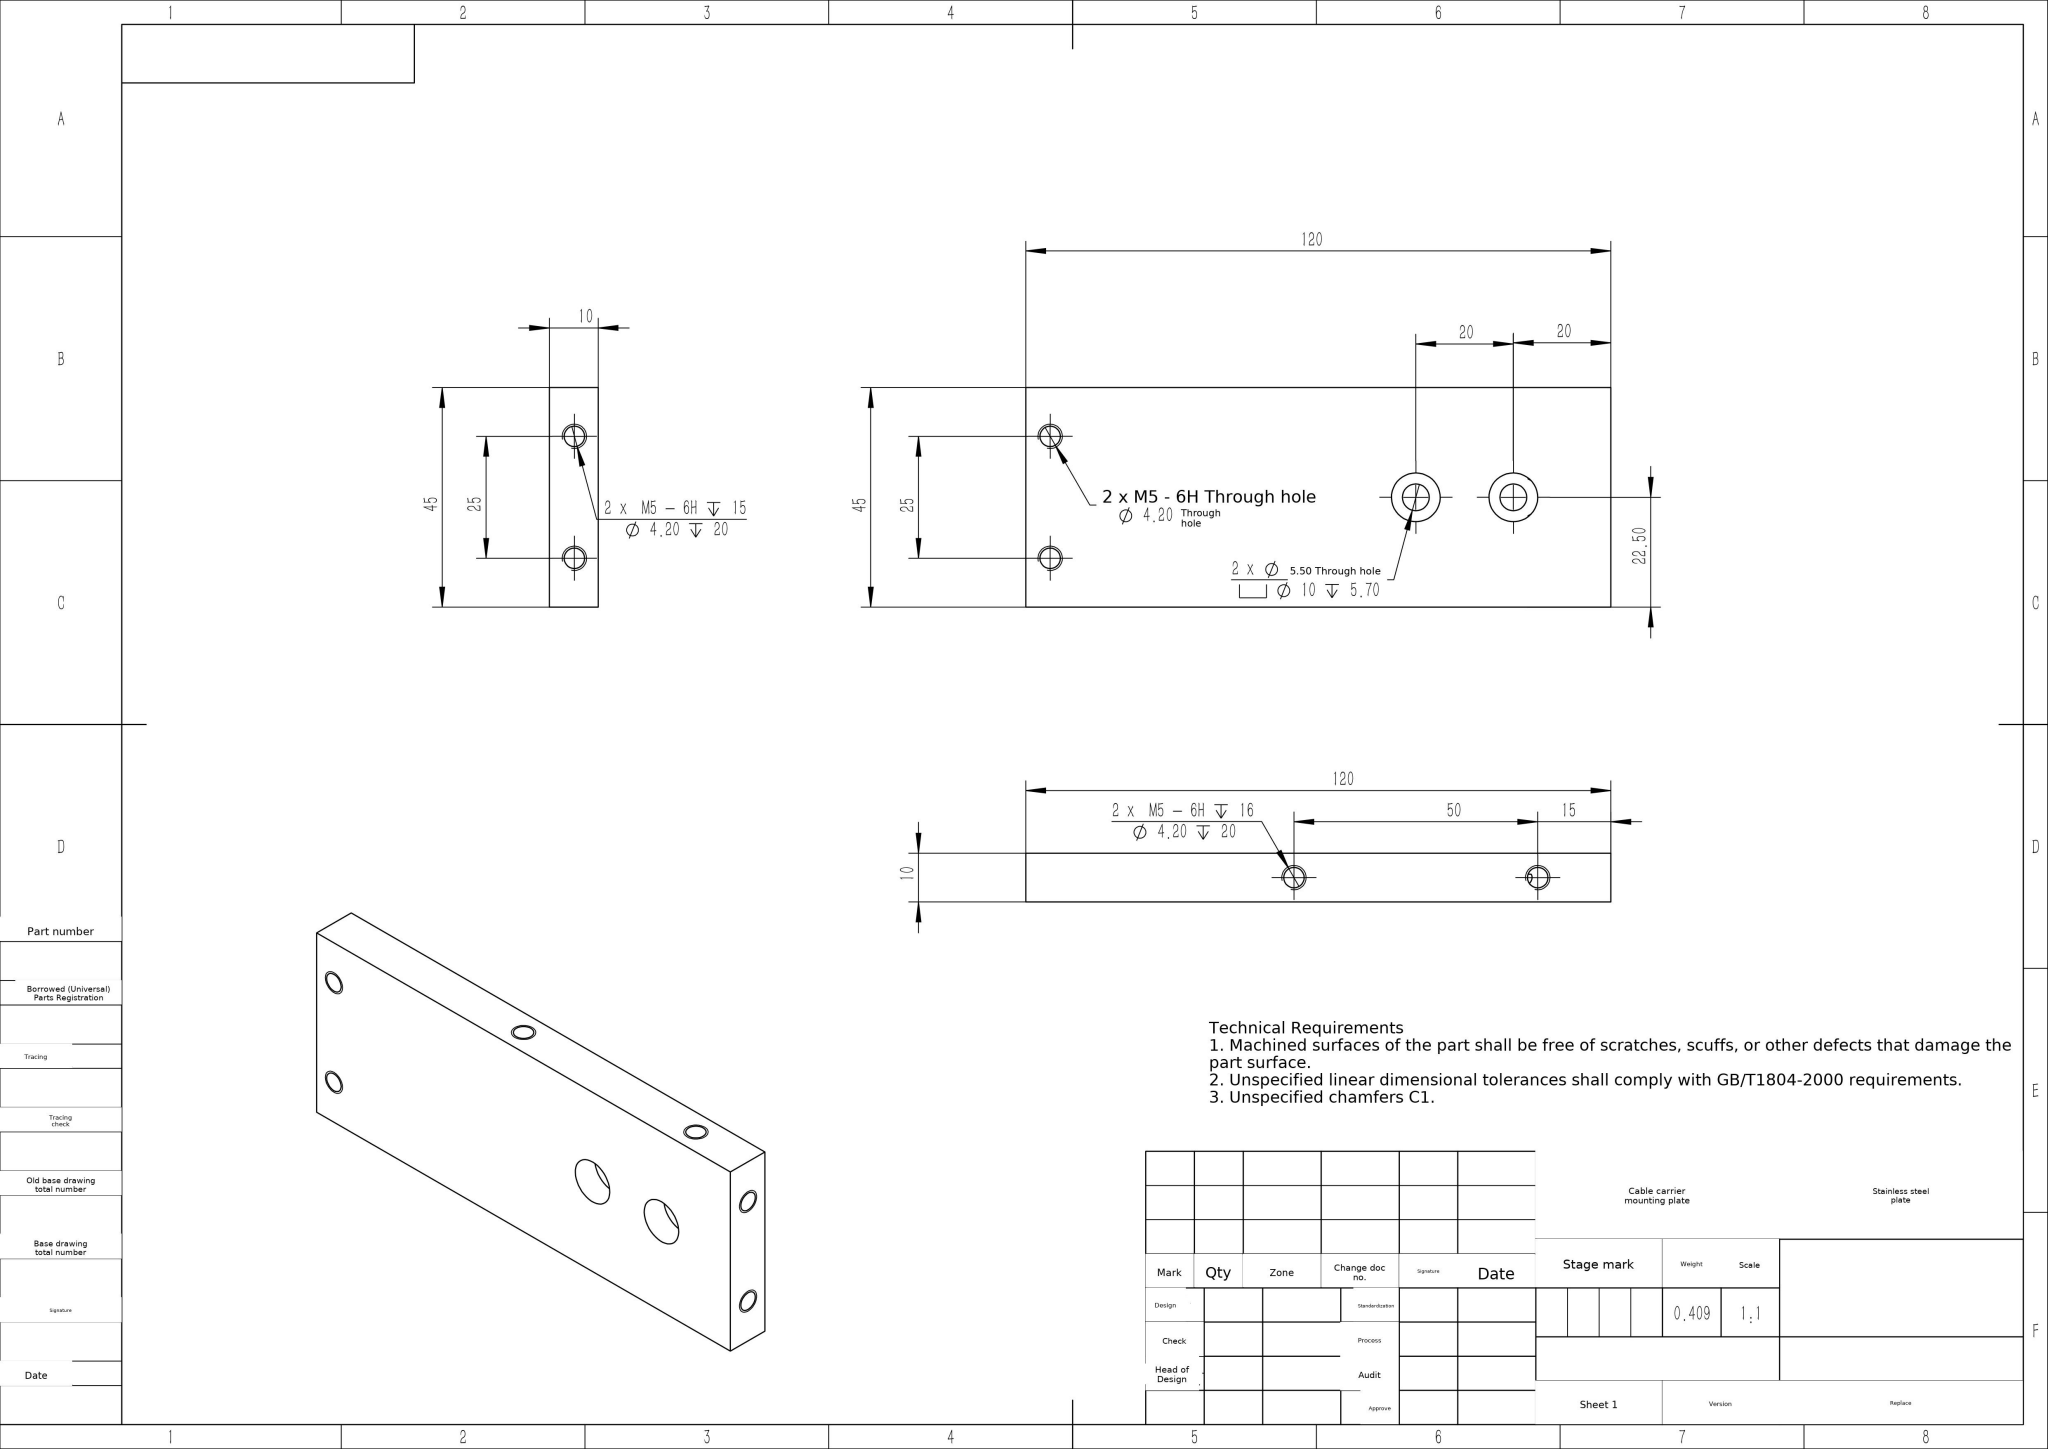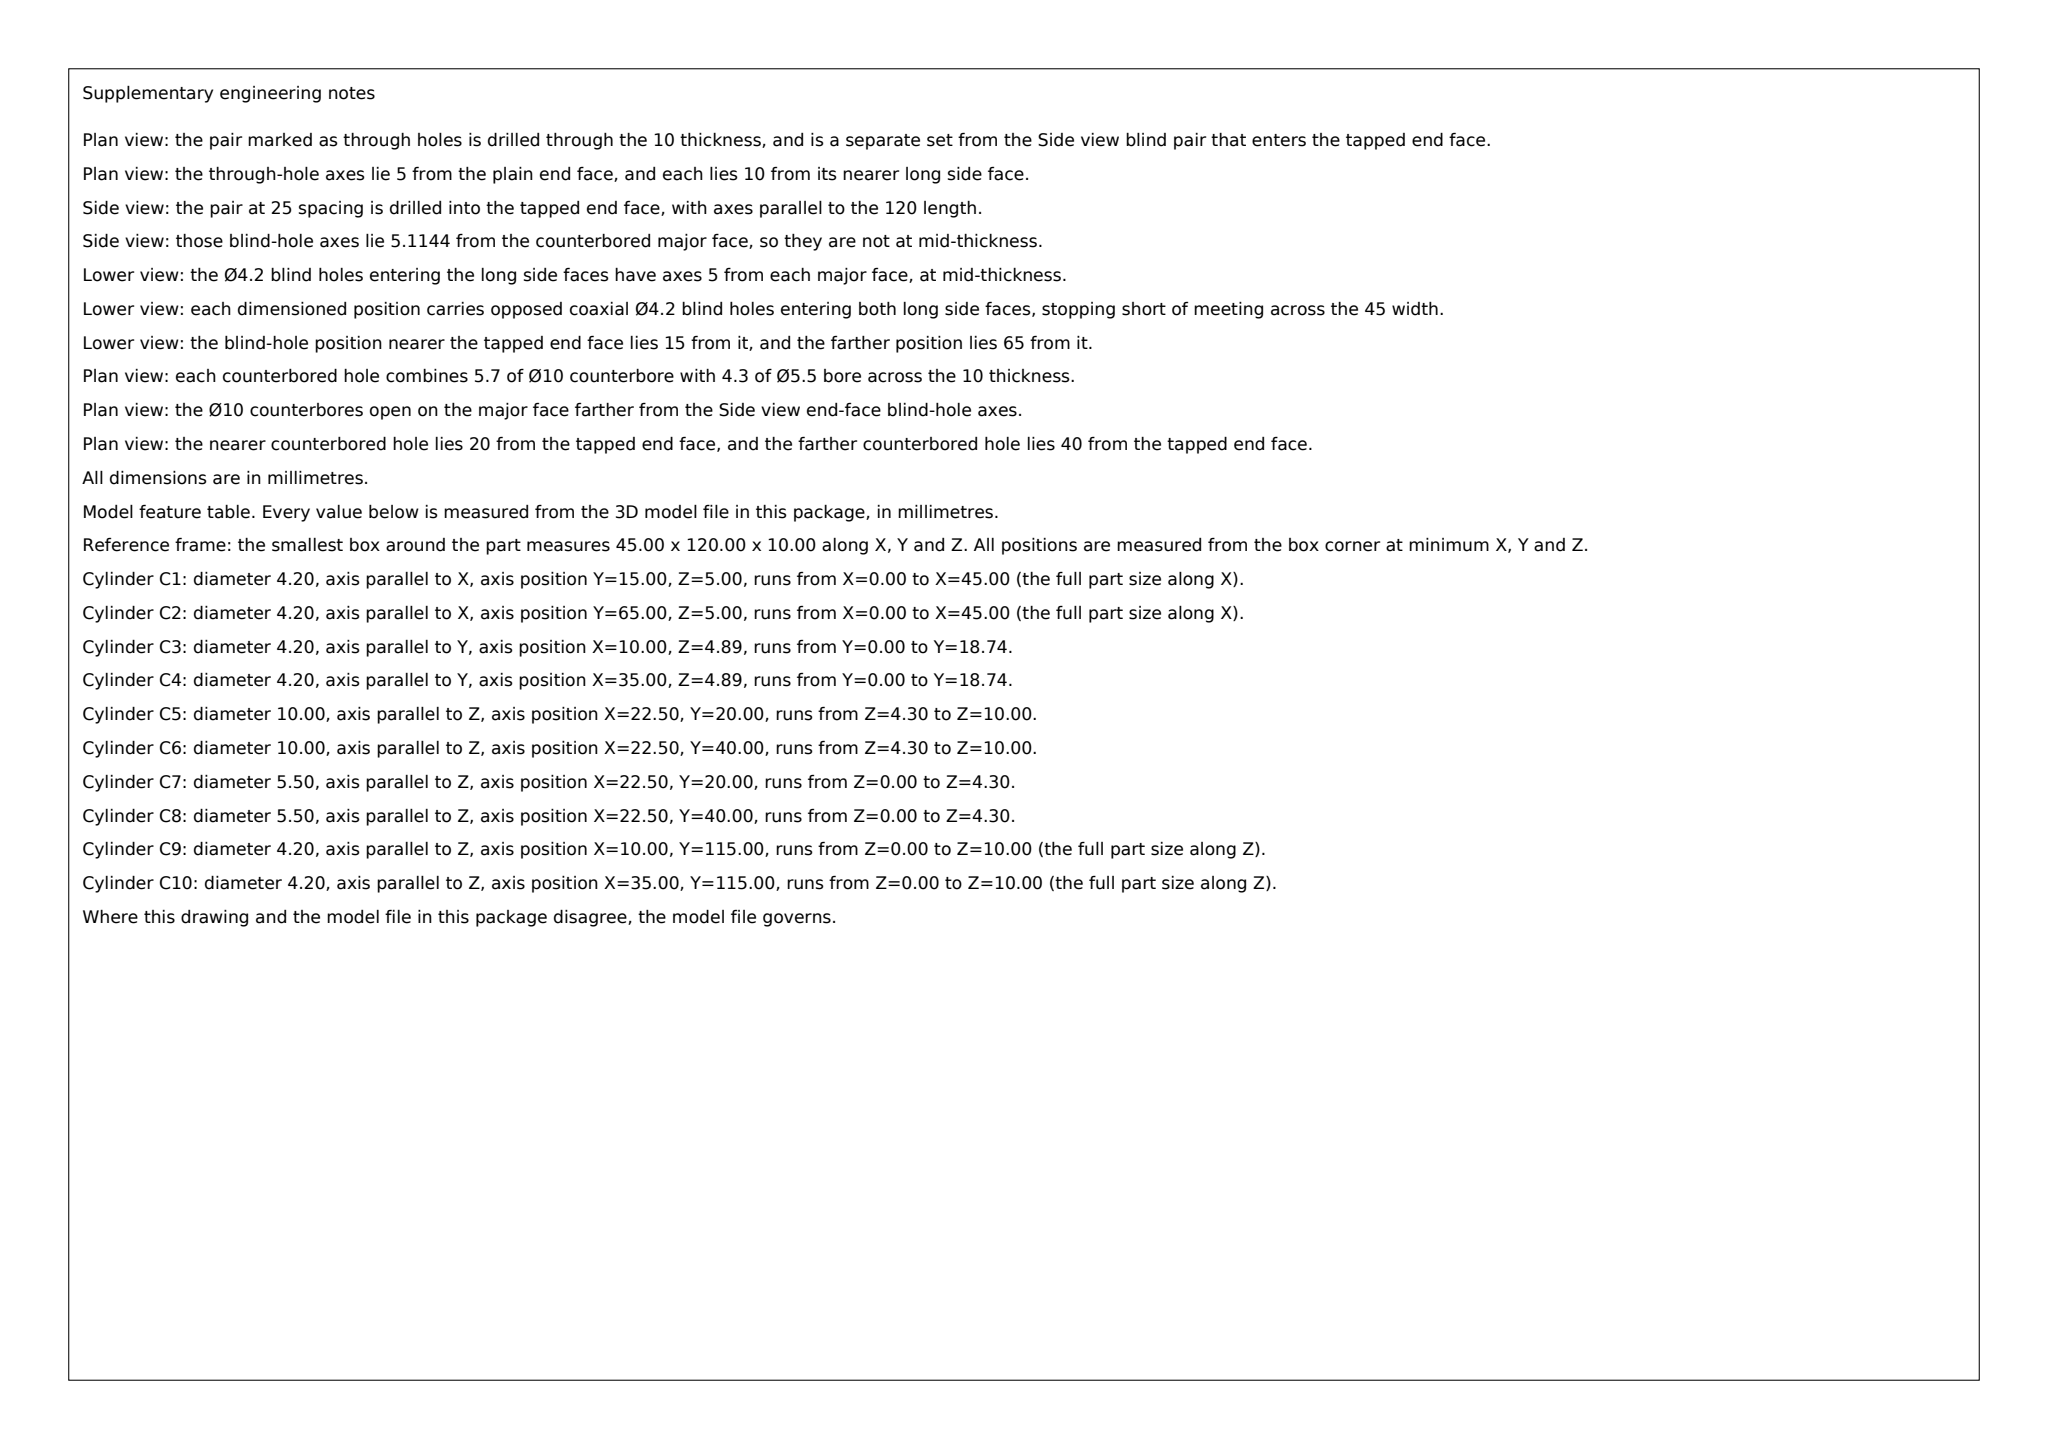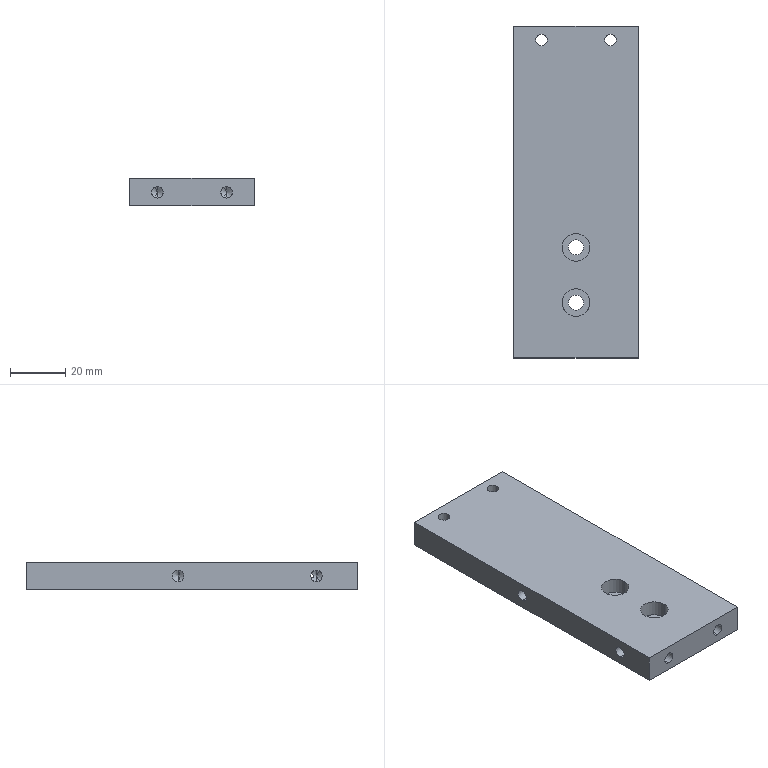Part | SolidWorks | mm | material Stainless steel plate | 1 solid | 44 faces | box 45 x 120 x 10 mm | volume 51129 mm3 | cylinder 24 | cone 12 | plane 8 | commonest cylinder face diameters 4.2 x16 5.5 x4 10 x4
Drawing notes:
OPP 120x10 FACE: 2 x M5-6H DP 16 / Ø4.20 DP 20, SAME LOCS AS SHOWN | from the solid: 4.2 dia holes, axis x, at y=15 & y=65, z=5, len 18.74 + 118 deg point; entering both x=0 and x=45 faces (4 total)
SIDE FACE TAPPED HOLES ON C/L OF 10 THK (5 FROM EA FACE) | from the solid: axis-x cylinders pos z=5.0 of 10.0 thk; y=15 & 65 (=15 & 65 from end, 50 apart)
build123d program:
from build123d import *

# Parameters (mm, degrees)
SKETCH6_W                                       = 45
SKETCH6_H                                       = 120
BOSS_EXTRUDE1_DEPTH                             = 10
M5_TAPPED_HOLE1_D                               = 4.2
M5_TAPPED_HOLE2_D                               = 4.2
M5_TAPPED_HOLE2_DEPTH                           = 18.738
M5_TAPPED_HOLE2_TIP                             = 1.262
M5_TAPPED_HOLE3_D                               = 4.2
M5_TAPPED_HOLE3_DEPTH                           = 18.738
M5_TAPPED_HOLE3_TIP                             = 1.262
M5_TAPPED_HOLE4_D                               = 4.2
M5_TAPPED_HOLE4_DEPTH                           = 18.738
M5_TAPPED_HOLE4_TIP                             = 1.262
M5_HEX_SOCKET_HEAD_CAP_SCREW_CBORE1_D           = 5.5
M5_HEX_SOCKET_HEAD_CAP_SCREW_CBORE1_CBORE_D     = 10
M5_HEX_SOCKET_HEAD_CAP_SCREW_CBORE1_CBORE_DEPTH = 5.7


with BuildPart() as part:
    # Sketch6 → Boss-Extrude1 (new body)
    with BuildSketch(Plane.XY):
        Rectangle(SKETCH6_W, SKETCH6_H)
    extrude(amount=BOSS_EXTRUDE1_DEPTH)

    # M5 Tapped Hole1 (through all)
    with Locations(Plane.XY.offset(10)):
        with Locations((12.5, 55), (-12.5, 55)):
            Hole(M5_TAPPED_HOLE1_D / 2)

    # M5 Tapped Hole2
    with Locations(Plane.ZY.offset(22.5)):
        with Locations((5, -45), (5, 5)):
            Hole(M5_TAPPED_HOLE2_D / 2, depth=M5_TAPPED_HOLE2_DEPTH)
            with Locations((0, 0, -(M5_TAPPED_HOLE2_DEPTH + M5_TAPPED_HOLE2_TIP / 2))):  # 118° drill point
                Cone(0, M5_TAPPED_HOLE2_D / 2, M5_TAPPED_HOLE2_TIP, mode=Mode.SUBTRACT)

    # M5 Tapped Hole3
    with Locations(Plane(origin=(22.5, 0, 0), x_dir=(0, 0, -1), z_dir=(1, 0, 0))):
        with Locations((-5, -45), (-5, 5)):
            Hole(M5_TAPPED_HOLE3_D / 2, depth=M5_TAPPED_HOLE3_DEPTH)
            with Locations((0, 0, -(M5_TAPPED_HOLE3_DEPTH + M5_TAPPED_HOLE3_TIP / 2))):  # 118° drill point
                Cone(0, M5_TAPPED_HOLE3_D / 2, M5_TAPPED_HOLE3_TIP, mode=Mode.SUBTRACT)

    # M5 Tapped Hole4
    with Locations(Plane(origin=(0, -60, 0), x_dir=(-1, 0, 0), z_dir=(0, -1, 0))):
        with Locations((12.5, -4.886), (-12.5, -4.886)):
            Hole(M5_TAPPED_HOLE4_D / 2, depth=M5_TAPPED_HOLE4_DEPTH)
            with Locations((0, 0, -(M5_TAPPED_HOLE4_DEPTH + M5_TAPPED_HOLE4_TIP / 2))):  # 118° drill point
                Cone(0, M5_TAPPED_HOLE4_D / 2, M5_TAPPED_HOLE4_TIP, mode=Mode.SUBTRACT)

    # M5 Hex Socket Head Cap Screw CBORE1 (through all)
    with Locations(Plane.XY.offset(10)):
        with Locations((0, -40), (0, -20)):
            CounterBoreHole(M5_HEX_SOCKET_HEAD_CAP_SCREW_CBORE1_D / 2, M5_HEX_SOCKET_HEAD_CAP_SCREW_CBORE1_CBORE_D / 2, M5_HEX_SOCKET_HEAD_CAP_SCREW_CBORE1_CBORE_DEPTH)


solid = part.part